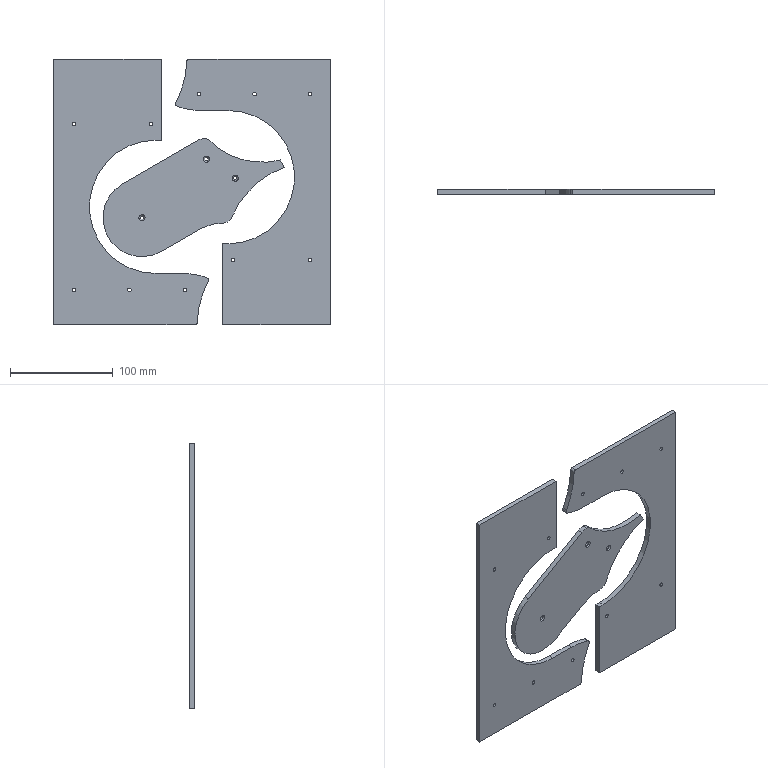CAM job | Mastercam | mm | 4 operations | part box 270 x 5 x 259
1. Contour (Ramp) | 3 - 3 平铣刀
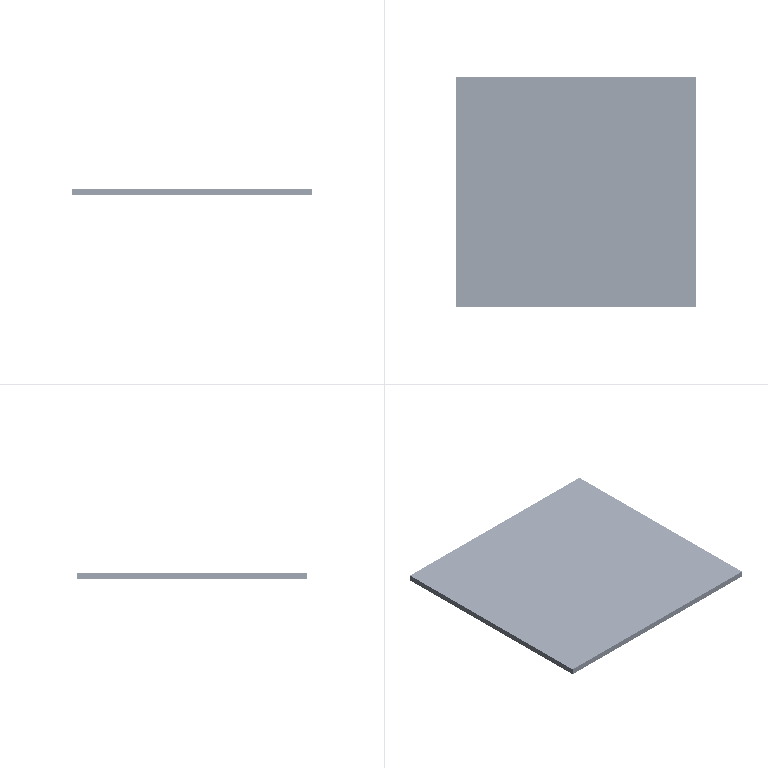2. Contour (2D) | 3 - 3 平铣刀
3. Drill/Counterbore | 7 - 4 倒角刀
4. Contour (2D chamfer) | 7 - 4 倒角刀